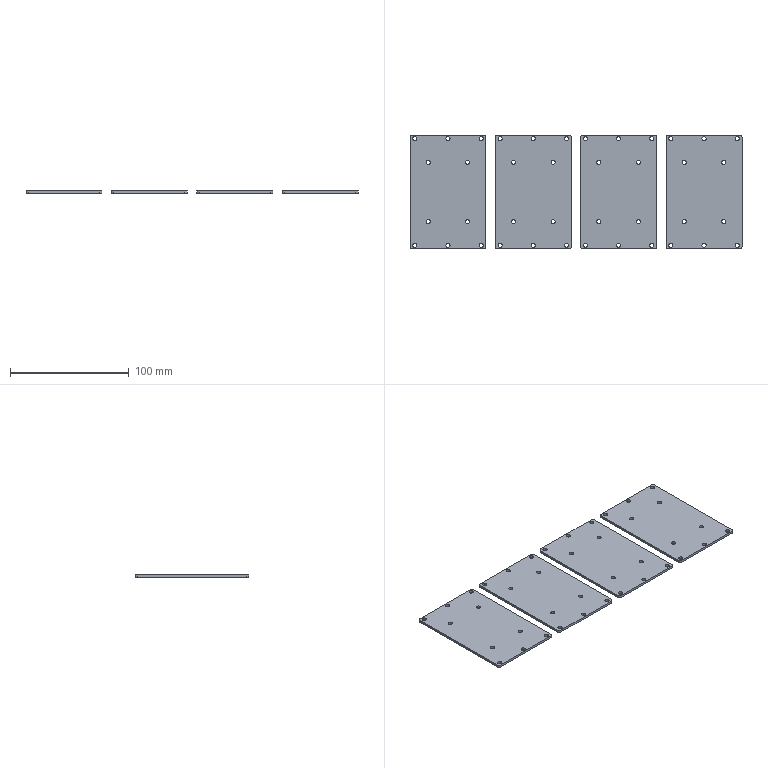CAM job | Mastercam | mm | 4 operations | part box 280 x 96 x 2
1. Contour (Ramp) | 3 - 3 平铣刀
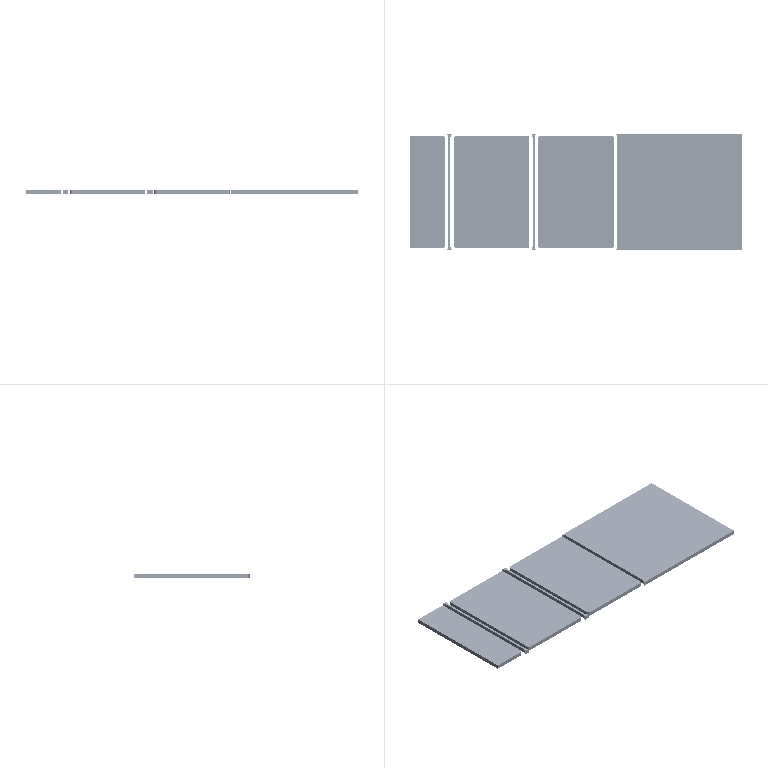2. Contour (2D) | 2 - 2 平铣刀
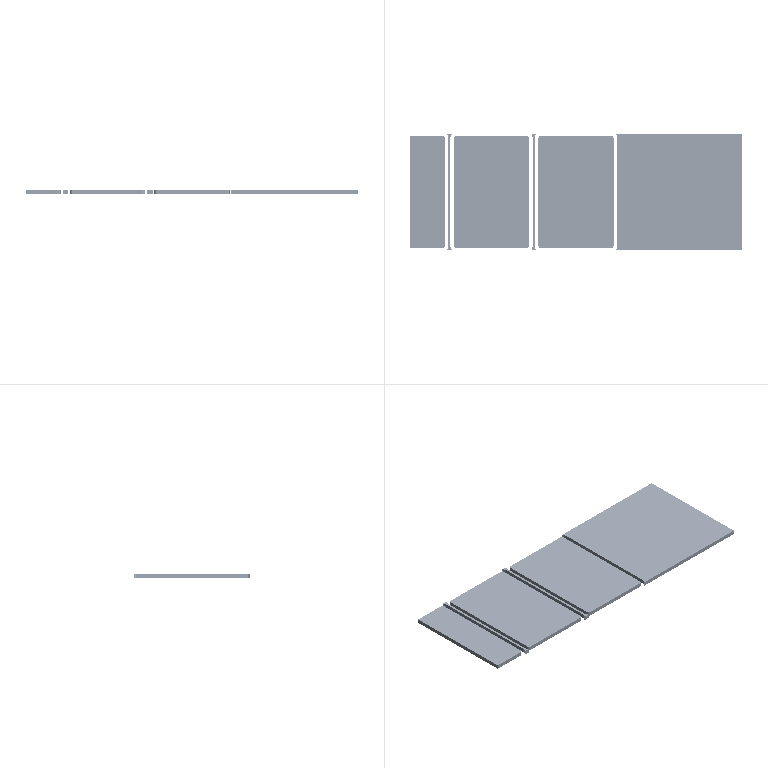3. Drill/Counterbore | 5 - 4 倒角刀
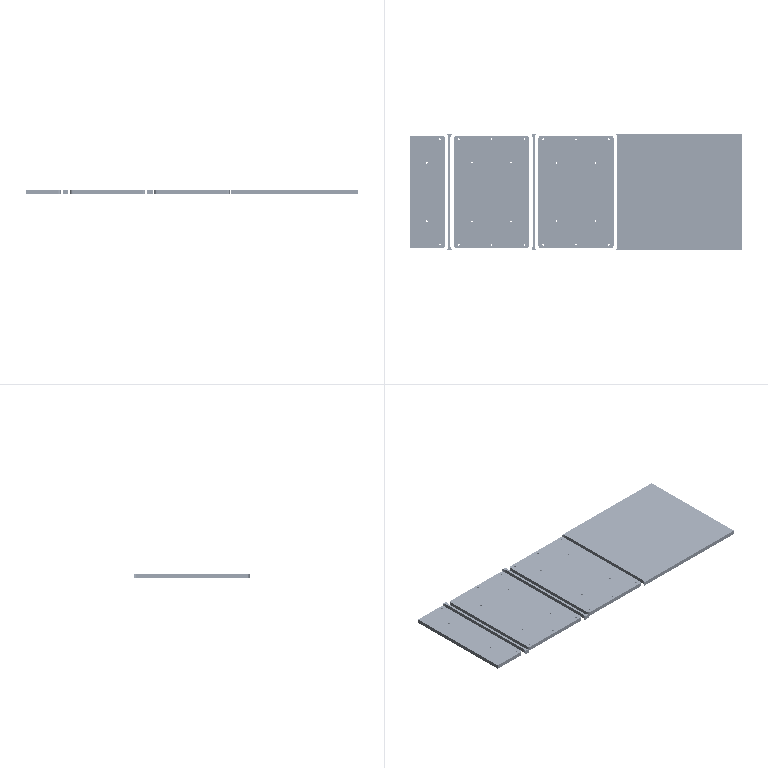4. Contour (2D chamfer) | 5 - 4 倒角刀